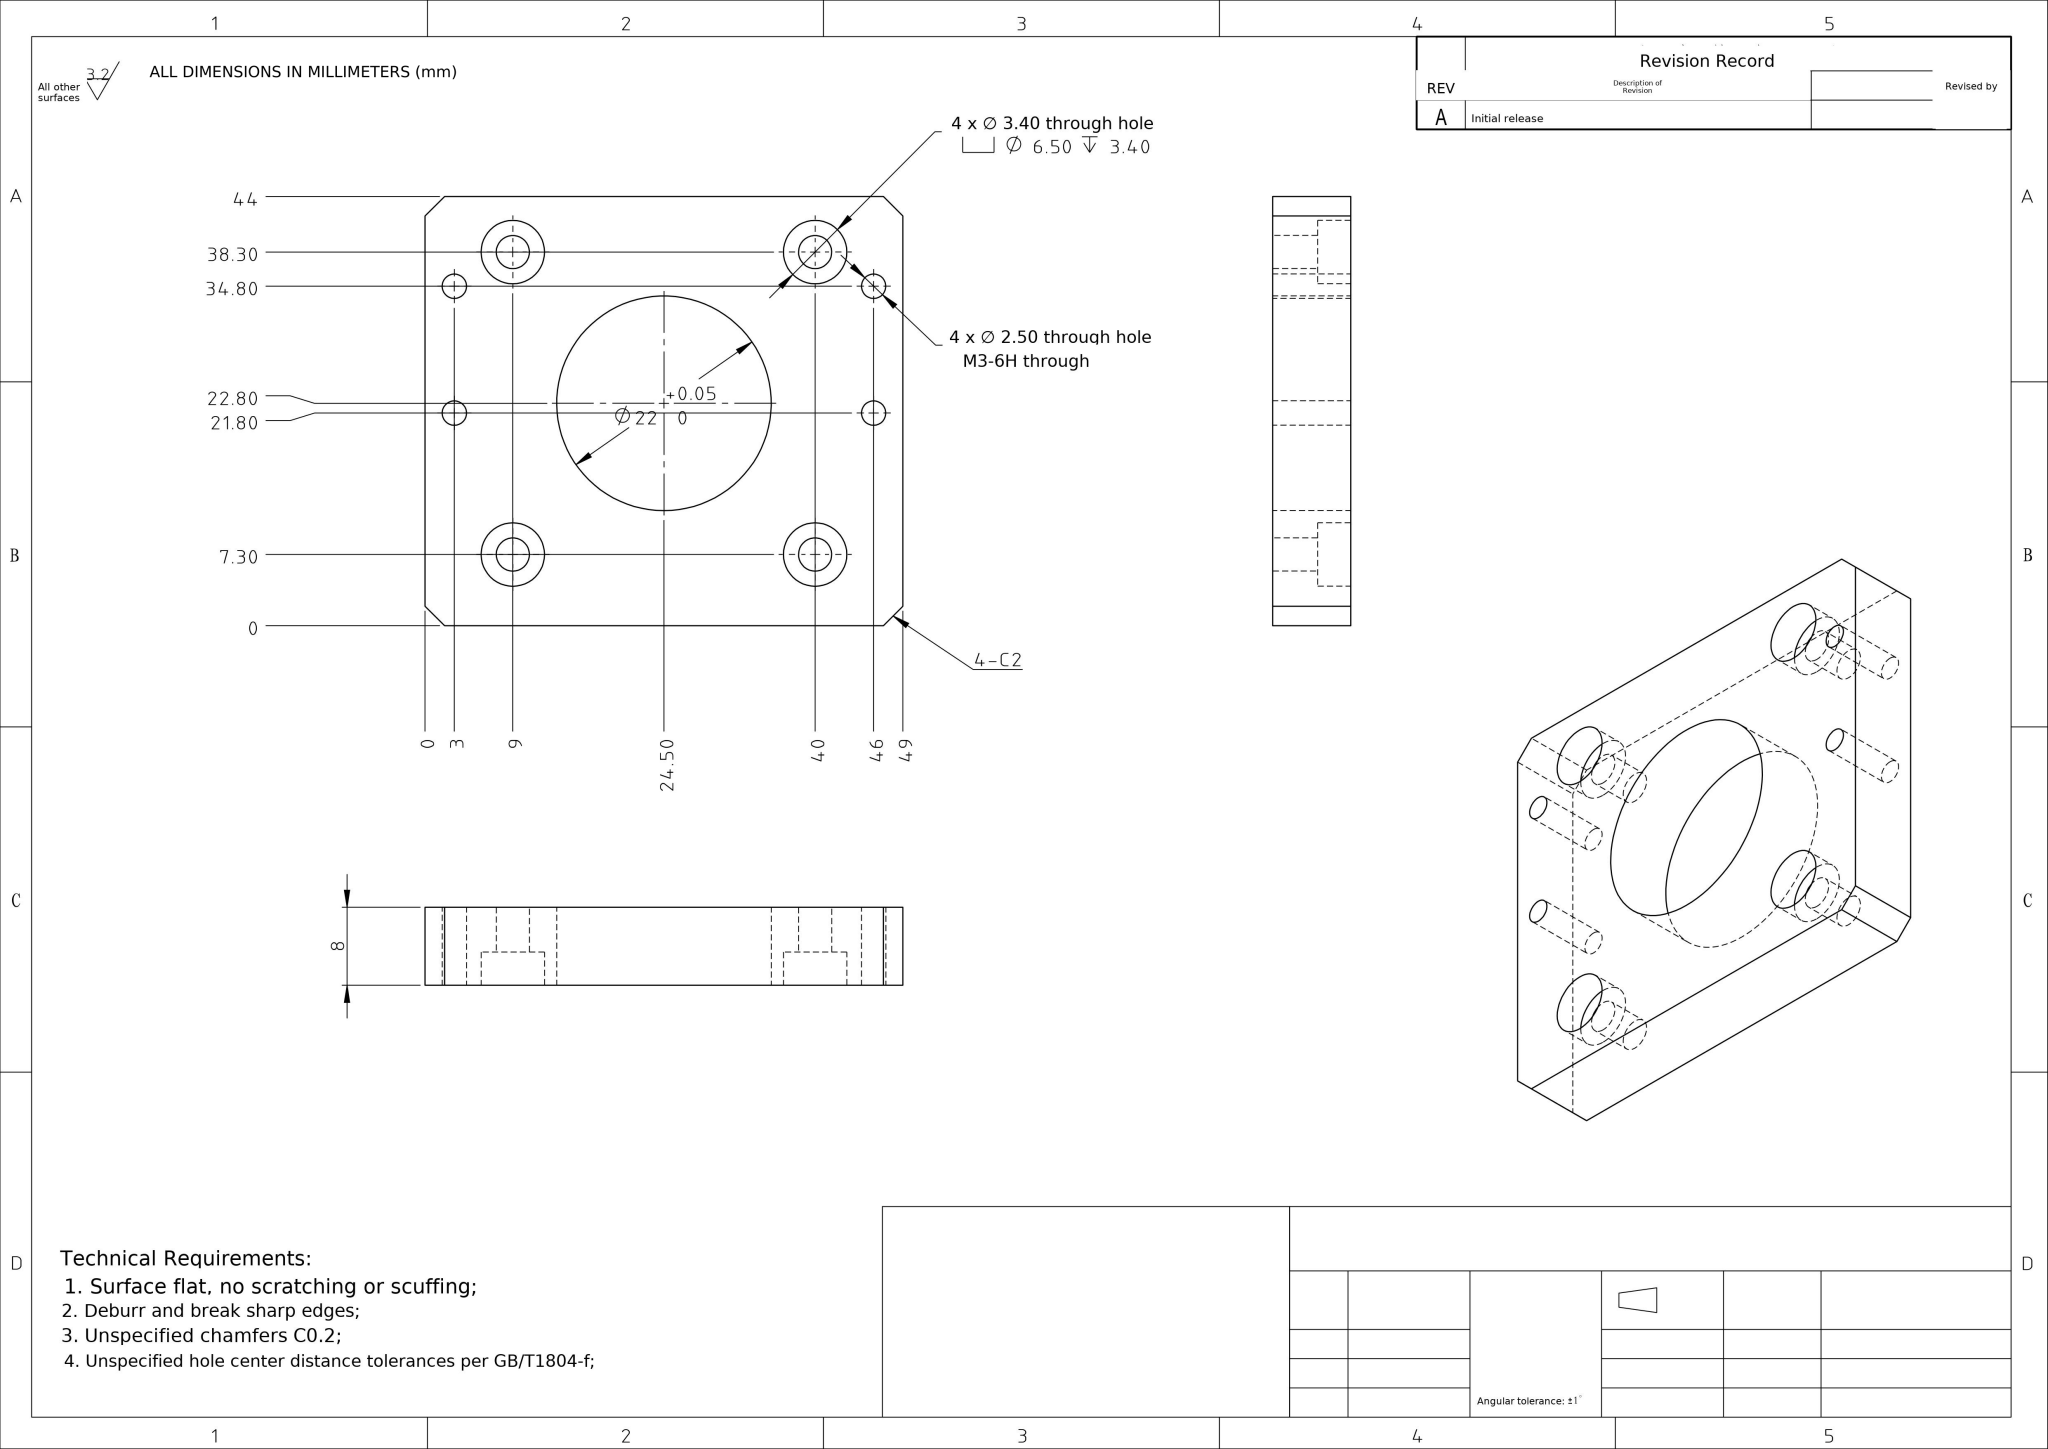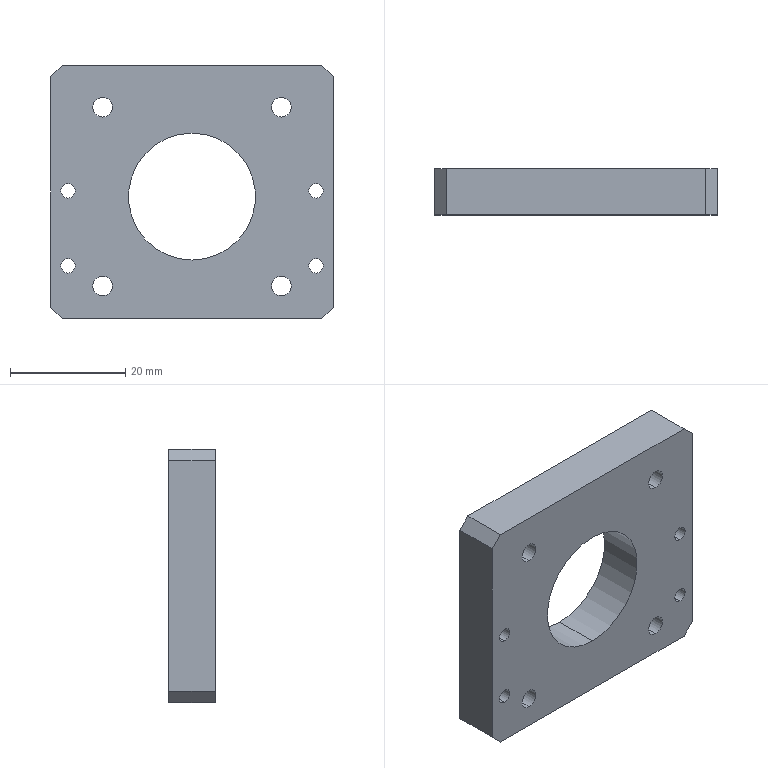Part | NX | mm | 1 solid | 40 faces | box 49 x 8 x 44 mm | volume 13368 mm3 | cylinder 26 | plane 14 | commonest cylinder face diameters 6.5 x8 3.4 x8 2.5 x8 22 x2